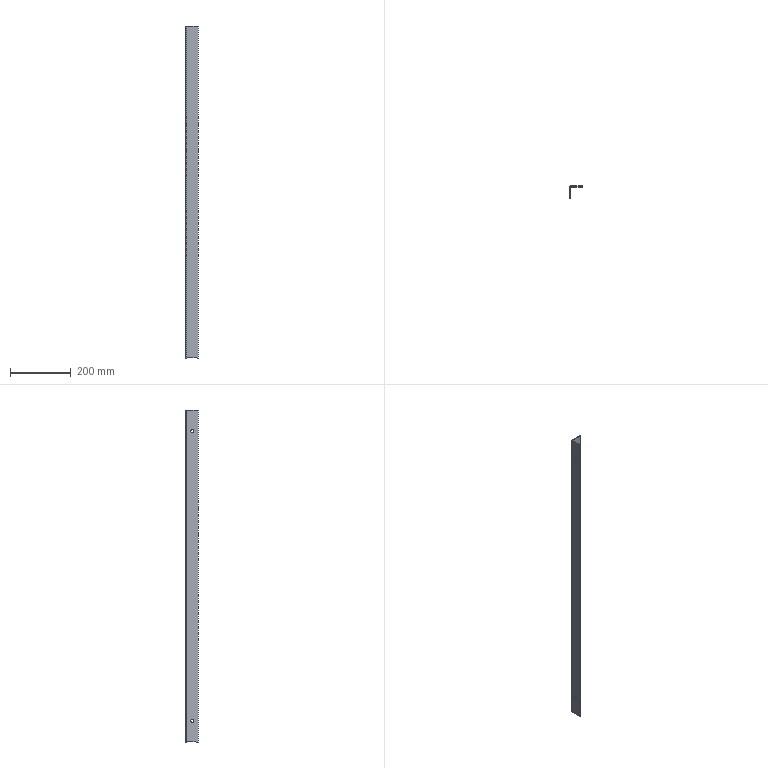Component | SolidWorks | CabinetWelding-1_MountingBeam-2 | 1 solid | 18 faces | box 40 x 40 x 1090 mm | volume 249073 mm3 | plane 12 | cylinder 6 | commonest cylinder face diameters 10 x4 6.2 x1 0.2 x1
STEP:
#1=COLOUR_RGB('',0.7922,0.8196,0.9333);
#2=FILL_AREA_STYLE_COLOUR('',#1);
#3=FILL_AREA_STYLE('',(#2));
#4=SURFACE_STYLE_FILL_AREA(#3);
#5=SURFACE_SIDE_STYLE('',(#4));
#6=SURFACE_STYLE_USAGE(.BOTH.,#5);
#7=PRESENTATION_STYLE_ASSIGNMENT((#6));
#8=CARTESIAN_POINT('',(18.936,29.641,55.907));
#9=VERTEX_POINT('',#8);
#10=CARTESIAN_POINT('',(18.936,29.641,56.301));
#11=VERTEX_POINT('',#10);
#12=CARTESIAN_POINT('',(18.936,29.641,56.104));
#13=DIRECTION('',(-1.,0.,0.));
#14=DIRECTION('',(0.,0.,1.));
#15=AXIS2_PLACEMENT_3D('',#12,#13,#14);
#16=CIRCLE('',#15,0.1969);
#17=EDGE_CURVE('',#9,#11,#16,.T.);
#18=ORIENTED_EDGE('',*,*,#17,.F.);
#19=CARTESIAN_POINT('',(18.818,29.641,55.907));
#20=VERTEX_POINT('',#19);
#21=CARTESIAN_POINT('',(19.212,29.641,55.907));
#22=DIRECTION('',(-1.,0.,0.));
#23=VECTOR('',#22,39.37);
#24=LINE('',#21,#23);
#25=EDGE_CURVE('',#9,#20,#24,.T.);
#26=ORIENTED_EDGE('',*,*,#25,.T.);
#27=CARTESIAN_POINT('',(18.818,29.641,56.301));
#28=VERTEX_POINT('',#27);
#29=CARTESIAN_POINT('',(18.818,29.641,56.104));
#30=DIRECTION('',(-1.,0.,0.));
#31=DIRECTION('',(0.,0.,1.));
#32=AXIS2_PLACEMENT_3D('',#29,#30,#31);
#33=CIRCLE('',#32,0.1969);
#34=EDGE_CURVE('',#20,#28,#33,.T.);
#35=ORIENTED_EDGE('',*,*,#34,.T.);
#36=CARTESIAN_POINT('',(19.212,29.641,56.301));
#37=DIRECTION('',(-1.,0.,0.));
#38=VECTOR('',#37,39.37);
#39=LINE('',#36,#38);
#40=EDGE_CURVE('',#11,#28,#39,.T.);
#41=ORIENTED_EDGE('',*,*,#40,.F.);
#42=EDGE_LOOP('',(#18,#26,#35,#41));
#43=FACE_OUTER_BOUND('',#42,.T.);
#44=CARTESIAN_POINT('',(19.212,29.641,56.104));
#45=DIRECTION('',(-1.,0.,0.));
#46=DIRECTION('',(0.,0.,1.));
#47=AXIS2_PLACEMENT_3D('',#44,#45,#46);
#48=CYLINDRICAL_SURFACE('',#47,0.1969);
#49=ADVANCED_FACE('',(#43),#48,.F.);
#50=CARTESIAN_POINT('',(18.936,29.641,93.309));
#51=VERTEX_POINT('',#50);
#52=CARTESIAN_POINT('',(18.936,29.641,93.703));
#53=VERTEX_POINT('',#52);
#54=CARTESIAN_POINT('',(18.936,29.641,93.506));
#55=DIRECTION('',(-1.,0.,0.));
#56=DIRECTION('',(0.,0.,1.));
#57=AXIS2_PLACEMENT_3D('',#54,#55,#56);
#58=CIRCLE('',#57,0.1969);
#59=EDGE_CURVE('',#51,#53,#58,.T.);
#60=ORIENTED_EDGE('',*,*,#59,.F.);
#61=CARTESIAN_POINT('',(18.818,29.641,93.309));
#62=VERTEX_POINT('',#61);
#63=CARTESIAN_POINT('',(19.212,29.641,93.309));
#64=DIRECTION('',(-1.,0.,0.));
#65=VECTOR('',#64,39.37);
#66=LINE('',#63,#65);
#67=EDGE_CURVE('',#51,#62,#66,.T.);
#68=ORIENTED_EDGE('',*,*,#67,.T.);
#69=CARTESIAN_POINT('',(18.818,29.641,93.703));
#70=VERTEX_POINT('',#69);
#71=CARTESIAN_POINT('',(18.818,29.641,93.506));
#72=DIRECTION('',(-1.,0.,0.));
#73=DIRECTION('',(0.,0.,1.));
#74=AXIS2_PLACEMENT_3D('',#71,#72,#73);
#75=CIRCLE('',#74,0.1969);
#76=EDGE_CURVE('',#62,#70,#75,.T.);
#77=ORIENTED_EDGE('',*,*,#76,.T.);
#78=CARTESIAN_POINT('',(19.212,29.641,93.703));
#79=DIRECTION('',(-1.,0.,0.));
#80=VECTOR('',#79,39.37);
#81=LINE('',#78,#80);
#82=EDGE_CURVE('',#53,#70,#81,.T.);
#83=ORIENTED_EDGE('',*,*,#82,.F.);
#84=EDGE_LOOP('',(#60,#68,#77,#83));
#85=FACE_OUTER_BOUND('',#84,.T.);
#86=CARTESIAN_POINT('',(19.212,29.641,93.506));
#87=DIRECTION('',(-1.,0.,0.));
#88=DIRECTION('',(0.,0.,1.));
#89=AXIS2_PLACEMENT_3D('',#86,#87,#88);
#90=CYLINDRICAL_SURFACE('',#89,0.1969);
#91=ADVANCED_FACE('',(#85),#90,.F.);
#92=CARTESIAN_POINT('',(18.936,28.893,96.26));
#93=VERTEX_POINT('',#92);
#94=CARTESIAN_POINT('',(18.936,30.345,96.26));
#95=VERTEX_POINT('',#94);
#96=CARTESIAN_POINT('',(18.936,30.467,96.26));
#97=DIRECTION('',(0.,1.,0.));
#98=VECTOR('',#97,39.37);
#99=LINE('',#96,#98);
#100=EDGE_CURVE('',#93,#95,#99,.T.);
#101=ORIENTED_EDGE('',*,*,#100,.T.);
#102=CARTESIAN_POINT('',(18.818,30.345,96.26));
#103=VERTEX_POINT('',#102);
#104=CARTESIAN_POINT('',(18.936,30.345,96.26));
#105=DIRECTION('',(-1.,0.,0.));
#106=VECTOR('',#105,39.37);
#107=LINE('',#104,#106);
#108=EDGE_CURVE('',#95,#103,#107,.T.);
#109=ORIENTED_EDGE('',*,*,#108,.T.);
#110=CARTESIAN_POINT('',(18.818,28.893,96.26));
#111=VERTEX_POINT('',#110);
#112=CARTESIAN_POINT('',(18.818,30.467,96.26));
#113=DIRECTION('',(0.,1.,0.));
#114=VECTOR('',#113,39.37);
#115=LINE('',#112,#114);
#116=EDGE_CURVE('',#111,#103,#115,.T.);
#117=ORIENTED_EDGE('',*,*,#116,.F.);
#118=CARTESIAN_POINT('',(18.936,28.893,96.26));
#119=DIRECTION('',(-1.,0.,0.));
#120=VECTOR('',#119,39.37);
#121=LINE('',#118,#120);
#122=EDGE_CURVE('',#93,#111,#121,.T.);
#123=ORIENTED_EDGE('',*,*,#122,.F.);
#124=EDGE_LOOP('',(#101,#109,#117,#123));
#125=FACE_OUTER_BOUND('',#124,.T.);
#126=CARTESIAN_POINT('',(18.936,30.467,96.26));
#127=DIRECTION('',(0.,-0.,1.));
#128=DIRECTION('',(1.,-0.,-0.));
#129=AXIS2_PLACEMENT_3D('',#126,#127,#128);
#130=PLANE('',#129);
#131=ADVANCED_FACE('',(#125),#130,.T.);
#132=CARTESIAN_POINT('',(18.936,29.641,56.104));
#133=DIRECTION('',(-1.,0.,0.));
#134=DIRECTION('',(0.,0.,1.));
#135=AXIS2_PLACEMENT_3D('',#132,#133,#134);
#136=CIRCLE('',#135,0.1969);
#137=EDGE_CURVE('',#11,#9,#136,.T.);
#138=ORIENTED_EDGE('',*,*,#137,.T.);
#139=ORIENTED_EDGE('',*,*,#17,.T.);
#140=EDGE_LOOP('',(#138,#139));
#141=FACE_BOUND('',#140,.T.);
#142=CARTESIAN_POINT('',(18.936,29.641,93.506));
#143=DIRECTION('',(-1.,0.,0.));
#144=DIRECTION('',(0.,0.,1.));
#145=AXIS2_PLACEMENT_3D('',#142,#143,#144);
#146=CIRCLE('',#145,0.1969);
#147=EDGE_CURVE('',#53,#51,#146,.T.);
#148=ORIENTED_EDGE('',*,*,#147,.T.);
#149=ORIENTED_EDGE('',*,*,#59,.T.);
#150=EDGE_LOOP('',(#148,#149));
#151=FACE_BOUND('',#150,.T.);
#152=CARTESIAN_POINT('',(18.936,30.345,53.347));
#153=VERTEX_POINT('',#152);
#154=CARTESIAN_POINT('',(18.936,30.345,96.26));
#155=DIRECTION('',(-0.,0.,-1.));
#156=VECTOR('',#155,39.37);
#157=LINE('',#154,#156);
#158=EDGE_CURVE('',#95,#153,#157,.T.);
#159=ORIENTED_EDGE('',*,*,#158,.F.);
#160=ORIENTED_EDGE('',*,*,#100,.F.);
#161=CARTESIAN_POINT('',(18.936,28.893,53.347));
#162=VERTEX_POINT('',#161);
#163=CARTESIAN_POINT('',(18.936,28.893,53.347));
#164=DIRECTION('',(0.,-0.,1.));
#165=VECTOR('',#164,39.37);
#166=LINE('',#163,#165);
#167=EDGE_CURVE('',#162,#93,#166,.T.);
#168=ORIENTED_EDGE('',*,*,#167,.F.);
#169=CARTESIAN_POINT('',(18.936,30.467,53.347));
#170=DIRECTION('',(-0.,-1.,-0.));
#171=VECTOR('',#170,39.37);
#172=LINE('',#169,#171);
#173=EDGE_CURVE('',#153,#162,#172,.T.);
#174=ORIENTED_EDGE('',*,*,#173,.F.);
#175=EDGE_LOOP('',(#159,#160,#168,#174));
#176=FACE_OUTER_BOUND('',#175,.T.);
#177=CARTESIAN_POINT('',(18.936,28.797,55.429));
#178=DIRECTION('',(-1.,0.,0.));
#179=DIRECTION('',(0.,-0.,1.));
#180=AXIS2_PLACEMENT_3D('',#177,#178,#179);
#181=PLANE('',#180);
#182=ADVANCED_FACE('',(#141,#151,#176),#181,.F.);
#183=CARTESIAN_POINT('',(18.818,29.641,56.104));
#184=DIRECTION('',(-1.,0.,0.));
#185=DIRECTION('',(0.,0.,1.));
#186=AXIS2_PLACEMENT_3D('',#183,#184,#185);
#187=CIRCLE('',#186,0.1969);
#188=EDGE_CURVE('',#28,#20,#187,.T.);
#189=ORIENTED_EDGE('',*,*,#188,.F.);
#190=ORIENTED_EDGE('',*,*,#34,.F.);
#191=EDGE_LOOP('',(#189,#190));
#192=FACE_BOUND('',#191,.T.);
#193=CARTESIAN_POINT('',(18.818,29.641,93.506));
#194=DIRECTION('',(-1.,0.,0.));
#195=DIRECTION('',(0.,0.,1.));
#196=AXIS2_PLACEMENT_3D('',#193,#194,#195);
#197=CIRCLE('',#196,0.1969);
#198=EDGE_CURVE('',#70,#62,#197,.T.);
#199=ORIENTED_EDGE('',*,*,#198,.F.);
#200=ORIENTED_EDGE('',*,*,#76,.F.);
#201=EDGE_LOOP('',(#199,#200));
#202=FACE_BOUND('',#201,.T.);
#203=ORIENTED_EDGE('',*,*,#116,.T.);
#204=CARTESIAN_POINT('',(18.818,30.345,53.347));
#205=VERTEX_POINT('',#204);
#206=CARTESIAN_POINT('',(18.818,30.345,96.26));
#207=DIRECTION('',(-0.,0.,-1.));
#208=VECTOR('',#207,39.37);
#209=LINE('',#206,#208);
#210=EDGE_CURVE('',#103,#205,#209,.T.);
#211=ORIENTED_EDGE('',*,*,#210,.T.);
#212=CARTESIAN_POINT('',(18.818,28.893,53.347));
#213=VERTEX_POINT('',#212);
#214=CARTESIAN_POINT('',(18.818,30.467,53.347));
#215=DIRECTION('',(-0.,-1.,-0.));
#216=VECTOR('',#215,39.37);
#217=LINE('',#214,#216);
#218=EDGE_CURVE('',#205,#213,#217,.T.);
#219=ORIENTED_EDGE('',*,*,#218,.T.);
#220=CARTESIAN_POINT('',(18.818,28.893,53.347));
#221=DIRECTION('',(0.,-0.,1.));
#222=VECTOR('',#221,39.37);
#223=LINE('',#220,#222);
#224=EDGE_CURVE('',#213,#111,#223,.T.);
#225=ORIENTED_EDGE('',*,*,#224,.T.);
#226=EDGE_LOOP('',(#203,#211,#219,#225));
#227=FACE_OUTER_BOUND('',#226,.T.);
#228=CARTESIAN_POINT('',(18.818,28.797,55.429));
#229=DIRECTION('',(-1.,0.,0.));
#230=DIRECTION('',(0.,-0.,1.));
#231=AXIS2_PLACEMENT_3D('',#228,#229,#230);
#232=PLANE('',#231);
#233=ADVANCED_FACE('',(#192,#202,#227),#232,.T.);
#234=CARTESIAN_POINT('',(18.936,30.345,53.347));
#235=DIRECTION('',(-1.,0.,-0.));
#236=VECTOR('',#235,39.37);
#237=LINE('',#234,#236);
#238=EDGE_CURVE('',#153,#205,#237,.T.);
#239=ORIENTED_EDGE('',*,*,#238,.F.);
#240=ORIENTED_EDGE('',*,*,#173,.T.);
#241=CARTESIAN_POINT('',(18.936,28.893,53.347));
#242=DIRECTION('',(-1.,0.,0.));
#243=VECTOR('',#242,39.37);
#244=LINE('',#241,#243);
#245=EDGE_CURVE('',#162,#213,#244,.T.);
#246=ORIENTED_EDGE('',*,*,#245,.T.);
#247=ORIENTED_EDGE('',*,*,#218,.F.);
#248=EDGE_LOOP('',(#239,#240,#246,#247));
#249=FACE_OUTER_BOUND('',#248,.T.);
#250=CARTESIAN_POINT('',(18.936,30.467,53.347));
#251=DIRECTION('',(-0.,0.,-1.));
#252=DIRECTION('',(-0.,-1.,-0.));
#253=AXIS2_PLACEMENT_3D('',#250,#251,#252);
#254=PLANE('',#253);
#255=ADVANCED_FACE('',(#249),#254,.T.);
#256=ORIENTED_EDGE('',*,*,#224,.F.);
#257=ORIENTED_EDGE('',*,*,#245,.F.);
#258=ORIENTED_EDGE('',*,*,#167,.T.);
#259=ORIENTED_EDGE('',*,*,#122,.T.);
#260=EDGE_LOOP('',(#256,#257,#258,#259));
#261=FACE_OUTER_BOUND('',#260,.T.);
#262=CARTESIAN_POINT('',(18.936,28.893,53.347));
#263=DIRECTION('',(-0.,-1.,-0.));
#264=DIRECTION('',(1.,-0.,-0.));
#265=AXIS2_PLACEMENT_3D('',#262,#263,#264);
#266=PLANE('',#265);
#267=ADVANCED_FACE('',(#261),#266,.T.);
#268=CARTESIAN_POINT('',(18.94,30.349,53.347));
#269=VERTEX_POINT('',#268);
#270=CARTESIAN_POINT('',(18.94,30.467,53.347));
#271=VERTEX_POINT('',#270);
#272=CARTESIAN_POINT('',(18.94,30.467,53.347));
#273=DIRECTION('',(-0.,1.,0.));
#274=VECTOR('',#273,39.37);
#275=LINE('',#272,#274);
#276=EDGE_CURVE('',#269,#271,#275,.T.);
#277=ORIENTED_EDGE('',*,*,#276,.F.);
#278=CARTESIAN_POINT('',(18.94,30.345,53.347));
#279=DIRECTION('',(-0.,0.,-1.));
#280=DIRECTION('',(1.,0.,0.));
#281=AXIS2_PLACEMENT_3D('',#278,#279,#280);
#282=CIRCLE('',#281,0.003937);
#283=EDGE_CURVE('',#153,#269,#282,.T.);
#284=ORIENTED_EDGE('',*,*,#283,.F.);
#285=ORIENTED_EDGE('',*,*,#238,.T.);
#286=CARTESIAN_POINT('',(18.94,30.345,53.347));
#287=DIRECTION('',(-0.,0.,-1.));
#288=DIRECTION('',(1.,0.,0.));
#289=AXIS2_PLACEMENT_3D('',#286,#287,#288);
#290=CIRCLE('',#289,0.122);
#291=EDGE_CURVE('',#205,#271,#290,.T.);
#292=ORIENTED_EDGE('',*,*,#291,.T.);
#293=EDGE_LOOP('',(#277,#284,#285,#292));
#294=FACE_OUTER_BOUND('',#293,.T.);
#295=CARTESIAN_POINT('',(18.94,30.345,53.347));
#296=DIRECTION('',(-0.,0.,-1.));
#297=DIRECTION('',(-1.,0.,0.));
#298=AXIS2_PLACEMENT_3D('',#295,#296,#297);
#299=PLANE('',#298);
#300=ADVANCED_FACE('',(#294),#299,.T.);
#301=CARTESIAN_POINT('',(18.94,30.349,96.26));
#302=VERTEX_POINT('',#301);
#303=CARTESIAN_POINT('',(18.94,30.345,96.26));
#304=DIRECTION('',(0.,-0.,1.));
#305=DIRECTION('',(1.,0.,0.));
#306=AXIS2_PLACEMENT_3D('',#303,#304,#305);
#307=CIRCLE('',#306,0.003937);
#308=EDGE_CURVE('',#302,#95,#307,.T.);
#309=ORIENTED_EDGE('',*,*,#308,.F.);
#310=CARTESIAN_POINT('',(18.94,30.467,96.26));
#311=VERTEX_POINT('',#310);
#312=CARTESIAN_POINT('',(18.94,30.349,96.26));
#313=DIRECTION('',(-0.,1.,0.));
#314=VECTOR('',#313,39.37);
#315=LINE('',#312,#314);
#316=EDGE_CURVE('',#302,#311,#315,.T.);
#317=ORIENTED_EDGE('',*,*,#316,.T.);
#318=CARTESIAN_POINT('',(18.94,30.345,96.26));
#319=DIRECTION('',(0.,-0.,1.));
#320=DIRECTION('',(1.,0.,0.));
#321=AXIS2_PLACEMENT_3D('',#318,#319,#320);
#322=CIRCLE('',#321,0.122);
#323=EDGE_CURVE('',#311,#103,#322,.T.);
#324=ORIENTED_EDGE('',*,*,#323,.T.);
#325=ORIENTED_EDGE('',*,*,#108,.F.);
#326=EDGE_LOOP('',(#309,#317,#324,#325));
#327=FACE_OUTER_BOUND('',#326,.T.);
#328=CARTESIAN_POINT('',(18.94,30.345,96.26));
#329=DIRECTION('',(-0.,0.,-1.));
#330=DIRECTION('',(-1.,0.,0.));
#331=AXIS2_PLACEMENT_3D('',#328,#329,#330);
#332=PLANE('',#331);
#333=ADVANCED_FACE('',(#327),#332,.F.);
#334=ORIENTED_EDGE('',*,*,#210,.F.);
#335=ORIENTED_EDGE('',*,*,#323,.F.);
#336=CARTESIAN_POINT('',(18.94,30.467,55.429));
#337=DIRECTION('',(0.,-0.,1.));
#338=VECTOR('',#337,39.37);
#339=LINE('',#336,#338);
#340=EDGE_CURVE('',#271,#311,#339,.T.);
#341=ORIENTED_EDGE('',*,*,#340,.F.);
#342=ORIENTED_EDGE('',*,*,#291,.F.);
#343=EDGE_LOOP('',(#334,#335,#341,#342));
#344=FACE_OUTER_BOUND('',#343,.T.);
#345=CARTESIAN_POINT('',(18.94,30.345,96.26));
#346=DIRECTION('',(0.,-0.,1.));
#347=DIRECTION('',(0.,1.,0.));
#348=AXIS2_PLACEMENT_3D('',#345,#346,#347);
#349=CYLINDRICAL_SURFACE('',#348,0.122);
#350=ADVANCED_FACE('',(#344),#349,.T.);
#351=ORIENTED_EDGE('',*,*,#158,.T.);
#352=ORIENTED_EDGE('',*,*,#283,.T.);
#353=CARTESIAN_POINT('',(18.94,30.349,53.347));
#354=DIRECTION('',(0.,-0.,1.));
#355=VECTOR('',#354,39.37);
#356=LINE('',#353,#355);
#357=EDGE_CURVE('',#269,#302,#356,.T.);
#358=ORIENTED_EDGE('',*,*,#357,.T.);
#359=ORIENTED_EDGE('',*,*,#308,.T.);
#360=EDGE_LOOP('',(#351,#352,#358,#359));
#361=FACE_OUTER_BOUND('',#360,.T.);
#362=CARTESIAN_POINT('',(18.94,30.345,96.26));
#363=DIRECTION('',(0.,-0.,1.));
#364=DIRECTION('',(0.,1.,0.));
#365=AXIS2_PLACEMENT_3D('',#362,#363,#364);
#366=CYLINDRICAL_SURFACE('',#365,0.003937);
#367=ADVANCED_FACE('',(#361),#366,.F.);
#368=CARTESIAN_POINT('',(20.393,30.467,96.26));
#369=VERTEX_POINT('',#368);
#370=CARTESIAN_POINT('',(18.936,30.467,96.26));
#371=DIRECTION('',(-1.,0.,0.));
#372=VECTOR('',#371,39.37);
#373=LINE('',#370,#372);
#374=EDGE_CURVE('',#369,#311,#373,.T.);
#375=ORIENTED_EDGE('',*,*,#374,.T.);
#376=ORIENTED_EDGE('',*,*,#316,.F.);
#377=CARTESIAN_POINT('',(20.393,30.349,96.26));
#378=VERTEX_POINT('',#377);
#379=CARTESIAN_POINT('',(18.818,30.349,96.26));
#380=DIRECTION('',(-1.,0.,0.));
#381=VECTOR('',#380,39.37);
#382=LINE('',#379,#381);
#383=EDGE_CURVE('',#378,#302,#382,.T.);
#384=ORIENTED_EDGE('',*,*,#383,.F.);
#385=CARTESIAN_POINT('',(20.393,30.467,96.26));
#386=DIRECTION('',(-0.,-1.,-0.));
#387=VECTOR('',#386,39.37);
#388=LINE('',#385,#387);
#389=EDGE_CURVE('',#369,#378,#388,.T.);
#390=ORIENTED_EDGE('',*,*,#389,.F.);
#391=EDGE_LOOP('',(#375,#376,#384,#390));
#392=FACE_OUTER_BOUND('',#391,.T.);
#393=CARTESIAN_POINT('',(18.936,30.467,96.26));
#394=DIRECTION('',(0.,-0.,1.));
#395=DIRECTION('',(1.,-0.,-0.));
#396=AXIS2_PLACEMENT_3D('',#393,#394,#395);
#397=PLANE('',#396);
#398=ADVANCED_FACE('',(#392),#397,.T.);
#399=CARTESIAN_POINT('',(20.393,30.349,53.347));
#400=VERTEX_POINT('',#399);
#401=CARTESIAN_POINT('',(18.818,30.349,53.347));
#402=DIRECTION('',(1.,-0.,-0.));
#403=VECTOR('',#402,39.37);
#404=LINE('',#401,#403);
#405=EDGE_CURVE('',#269,#400,#404,.T.);
#406=ORIENTED_EDGE('',*,*,#405,.F.);
#407=ORIENTED_EDGE('',*,*,#276,.T.);
#408=CARTESIAN_POINT('',(20.393,30.467,53.347));
#409=VERTEX_POINT('',#408);
#410=CARTESIAN_POINT('',(20.393,30.467,53.347));
#411=DIRECTION('',(1.,-0.,-0.));
#412=VECTOR('',#411,39.37);
#413=LINE('',#410,#412);
#414=EDGE_CURVE('',#271,#409,#413,.T.);
#415=ORIENTED_EDGE('',*,*,#414,.T.);
#416=CARTESIAN_POINT('',(20.393,30.467,53.347));
#417=DIRECTION('',(-0.,-1.,-0.));
#418=VECTOR('',#417,39.37);
#419=LINE('',#416,#418);
#420=EDGE_CURVE('',#409,#400,#419,.T.);
#421=ORIENTED_EDGE('',*,*,#420,.T.);
#422=EDGE_LOOP('',(#406,#407,#415,#421));
#423=FACE_OUTER_BOUND('',#422,.T.);
#424=CARTESIAN_POINT('',(20.393,30.467,53.347));
#425=DIRECTION('',(-0.,0.,-1.));
#426=DIRECTION('',(-1.,0.,0.));
#427=AXIS2_PLACEMENT_3D('',#424,#425,#426);
#428=PLANE('',#427);
#429=ADVANCED_FACE('',(#423),#428,.T.);
#430=ORIENTED_EDGE('',*,*,#414,.F.);
#431=ORIENTED_EDGE('',*,*,#340,.T.);
#432=ORIENTED_EDGE('',*,*,#374,.F.);
#433=CARTESIAN_POINT('',(20.393,30.467,96.26));
#434=DIRECTION('',(0.,-0.,1.));
#435=VECTOR('',#434,39.37);
#436=LINE('',#433,#435);
#437=EDGE_CURVE('',#409,#369,#436,.T.);
#438=ORIENTED_EDGE('',*,*,#437,.F.);
#439=EDGE_LOOP('',(#430,#431,#432,#438));
#440=FACE_OUTER_BOUND('',#439,.T.);
#441=CARTESIAN_POINT('',(18.818,30.467,55.429));
#442=DIRECTION('',(0.,1.,0.));
#443=DIRECTION('',(-1.,0.,0.));
#444=AXIS2_PLACEMENT_3D('',#441,#442,#443);
#445=PLANE('',#444);
#446=ADVANCED_FACE('',(#440),#445,.T.);
#447=ORIENTED_EDGE('',*,*,#357,.F.);
#448=ORIENTED_EDGE('',*,*,#405,.T.);
#449=CARTESIAN_POINT('',(20.393,30.349,55.429));
#450=DIRECTION('',(0.,-0.,1.));
#451=VECTOR('',#450,39.37);
#452=LINE('',#449,#451);
#453=EDGE_CURVE('',#400,#378,#452,.T.);
#454=ORIENTED_EDGE('',*,*,#453,.T.);
#455=ORIENTED_EDGE('',*,*,#383,.T.);
#456=EDGE_LOOP('',(#447,#448,#454,#455));
#457=FACE_OUTER_BOUND('',#456,.T.);
#458=CARTESIAN_POINT('',(18.818,30.349,55.429));
#459=DIRECTION('',(0.,1.,0.));
#460=DIRECTION('',(-1.,0.,0.));
#461=AXIS2_PLACEMENT_3D('',#458,#459,#460);
#462=PLANE('',#461);
#463=ADVANCED_FACE('',(#457),#462,.F.);
#464=ORIENTED_EDGE('',*,*,#453,.F.);
#465=ORIENTED_EDGE('',*,*,#420,.F.);
#466=ORIENTED_EDGE('',*,*,#437,.T.);
#467=ORIENTED_EDGE('',*,*,#389,.T.);
#468=EDGE_LOOP('',(#464,#465,#466,#467));
#469=FACE_OUTER_BOUND('',#468,.T.);
#470=CARTESIAN_POINT('',(20.393,30.467,96.26));
#471=DIRECTION('',(1.,-0.,-0.));
#472=DIRECTION('',(0.,1.,0.));
#473=AXIS2_PLACEMENT_3D('',#470,#471,#472);
#474=PLANE('',#473);
#475=ADVANCED_FACE('',(#469),#474,.T.);
#476=ORIENTED_EDGE('',*,*,#67,.F.);
#477=ORIENTED_EDGE('',*,*,#147,.F.);
#478=ORIENTED_EDGE('',*,*,#82,.T.);
#479=ORIENTED_EDGE('',*,*,#198,.T.);
#480=EDGE_LOOP('',(#476,#477,#478,#479));
#481=FACE_OUTER_BOUND('',#480,.T.);
#482=CARTESIAN_POINT('',(19.212,29.641,93.506));
#483=DIRECTION('',(-1.,0.,0.));
#484=DIRECTION('',(0.,0.,1.));
#485=AXIS2_PLACEMENT_3D('',#482,#483,#484);
#486=CYLINDRICAL_SURFACE('',#485,0.1969);
#487=ADVANCED_FACE('',(#481),#486,.F.);
#488=ORIENTED_EDGE('',*,*,#25,.F.);
#489=ORIENTED_EDGE('',*,*,#137,.F.);
#490=ORIENTED_EDGE('',*,*,#40,.T.);
#491=ORIENTED_EDGE('',*,*,#188,.T.);
#492=EDGE_LOOP('',(#488,#489,#490,#491));
#493=FACE_OUTER_BOUND('',#492,.T.);
#494=CARTESIAN_POINT('',(19.212,29.641,56.104));
#495=DIRECTION('',(-1.,0.,0.));
#496=DIRECTION('',(0.,0.,1.));
#497=AXIS2_PLACEMENT_3D('',#494,#495,#496);
#498=CYLINDRICAL_SURFACE('',#497,0.1969);
#499=ADVANCED_FACE('',(#493),#498,.F.);
#500=CLOSED_SHELL('',(#49,#91,#131,#182,#233,#255,#267,#300,#333,#350,#367,#398,#429,#446,#463,#475,#487,#499));
#501=MANIFOLD_SOLID_BREP('',#500);
#502=STYLED_ITEM('',(#7),#501);
#503=PRESENTATION_LAYER_ASSIGNMENT('','',(#502));
#504=(LENGTH_UNIT()NAMED_UNIT(*)SI_UNIT($,.METRE.));
#505=LENGTH_MEASURE_WITH_UNIT(LENGTH_MEASURE(0.0254),#504);
#506=DIMENSIONAL_EXPONENTS(1.,0.,0.,0.,0.,0.,0.);
#507=(CONVERSION_BASED_UNIT('',#505)LENGTH_UNIT()NAMED_UNIT(#506));
#508=UNCERTAINTY_MEASURE_WITH_UNIT(LENGTH_MEASURE(0.00001),#507,'','');
#509=(NAMED_UNIT(*)PLANE_ANGLE_UNIT()SI_UNIT($,.RADIAN.));
#510=(NAMED_UNIT(*)SI_UNIT($,.STERADIAN.)SOLID_ANGLE_UNIT());
#511=(GEOMETRIC_REPRESENTATION_CONTEXT(3)GLOBAL_UNCERTAINTY_ASSIGNED_CONTEXT((#508))GLOBAL_UNIT_ASSIGNED_CONTEXT((#507,#509,#510))REPRESENTATION_CONTEXT('',''));
#512=MECHANICAL_DESIGN_GEOMETRIC_PRESENTATION_REPRESENTATION('',(#502),#511);
#513=CARTESIAN_POINT('',(0.,0.,0.));
#514=DIRECTION('',(0.,0.,1.));
#515=DIRECTION('',(1.,0.,0.));
#516=AXIS2_PLACEMENT_3D('',#513,#514,#515);
#517=(LENGTH_UNIT()NAMED_UNIT(*)SI_UNIT($,.METRE.));
#518=LENGTH_MEASURE_WITH_UNIT(LENGTH_MEASURE(0.0254),#517);
#519=DIMENSIONAL_EXPONENTS(1.,0.,0.,0.,0.,0.,0.);
#520=(CONVERSION_BASED_UNIT('',#518)LENGTH_UNIT()NAMED_UNIT(#519));
#521=UNCERTAINTY_MEASURE_WITH_UNIT(LENGTH_MEASURE(0.00001),#520,'','');
#522=(NAMED_UNIT(*)PLANE_ANGLE_UNIT()SI_UNIT($,.RADIAN.));
#523=(NAMED_UNIT(*)SI_UNIT($,.STERADIAN.)SOLID_ANGLE_UNIT());
#524=(GEOMETRIC_REPRESENTATION_CONTEXT(3)GLOBAL_UNCERTAINTY_ASSIGNED_CONTEXT((#521))GLOBAL_UNIT_ASSIGNED_CONTEXT((#520,#522,#523))REPRESENTATION_CONTEXT('',''));
#525=ADVANCED_BREP_SHAPE_REPRESENTATION('',(#501,#516),#524);